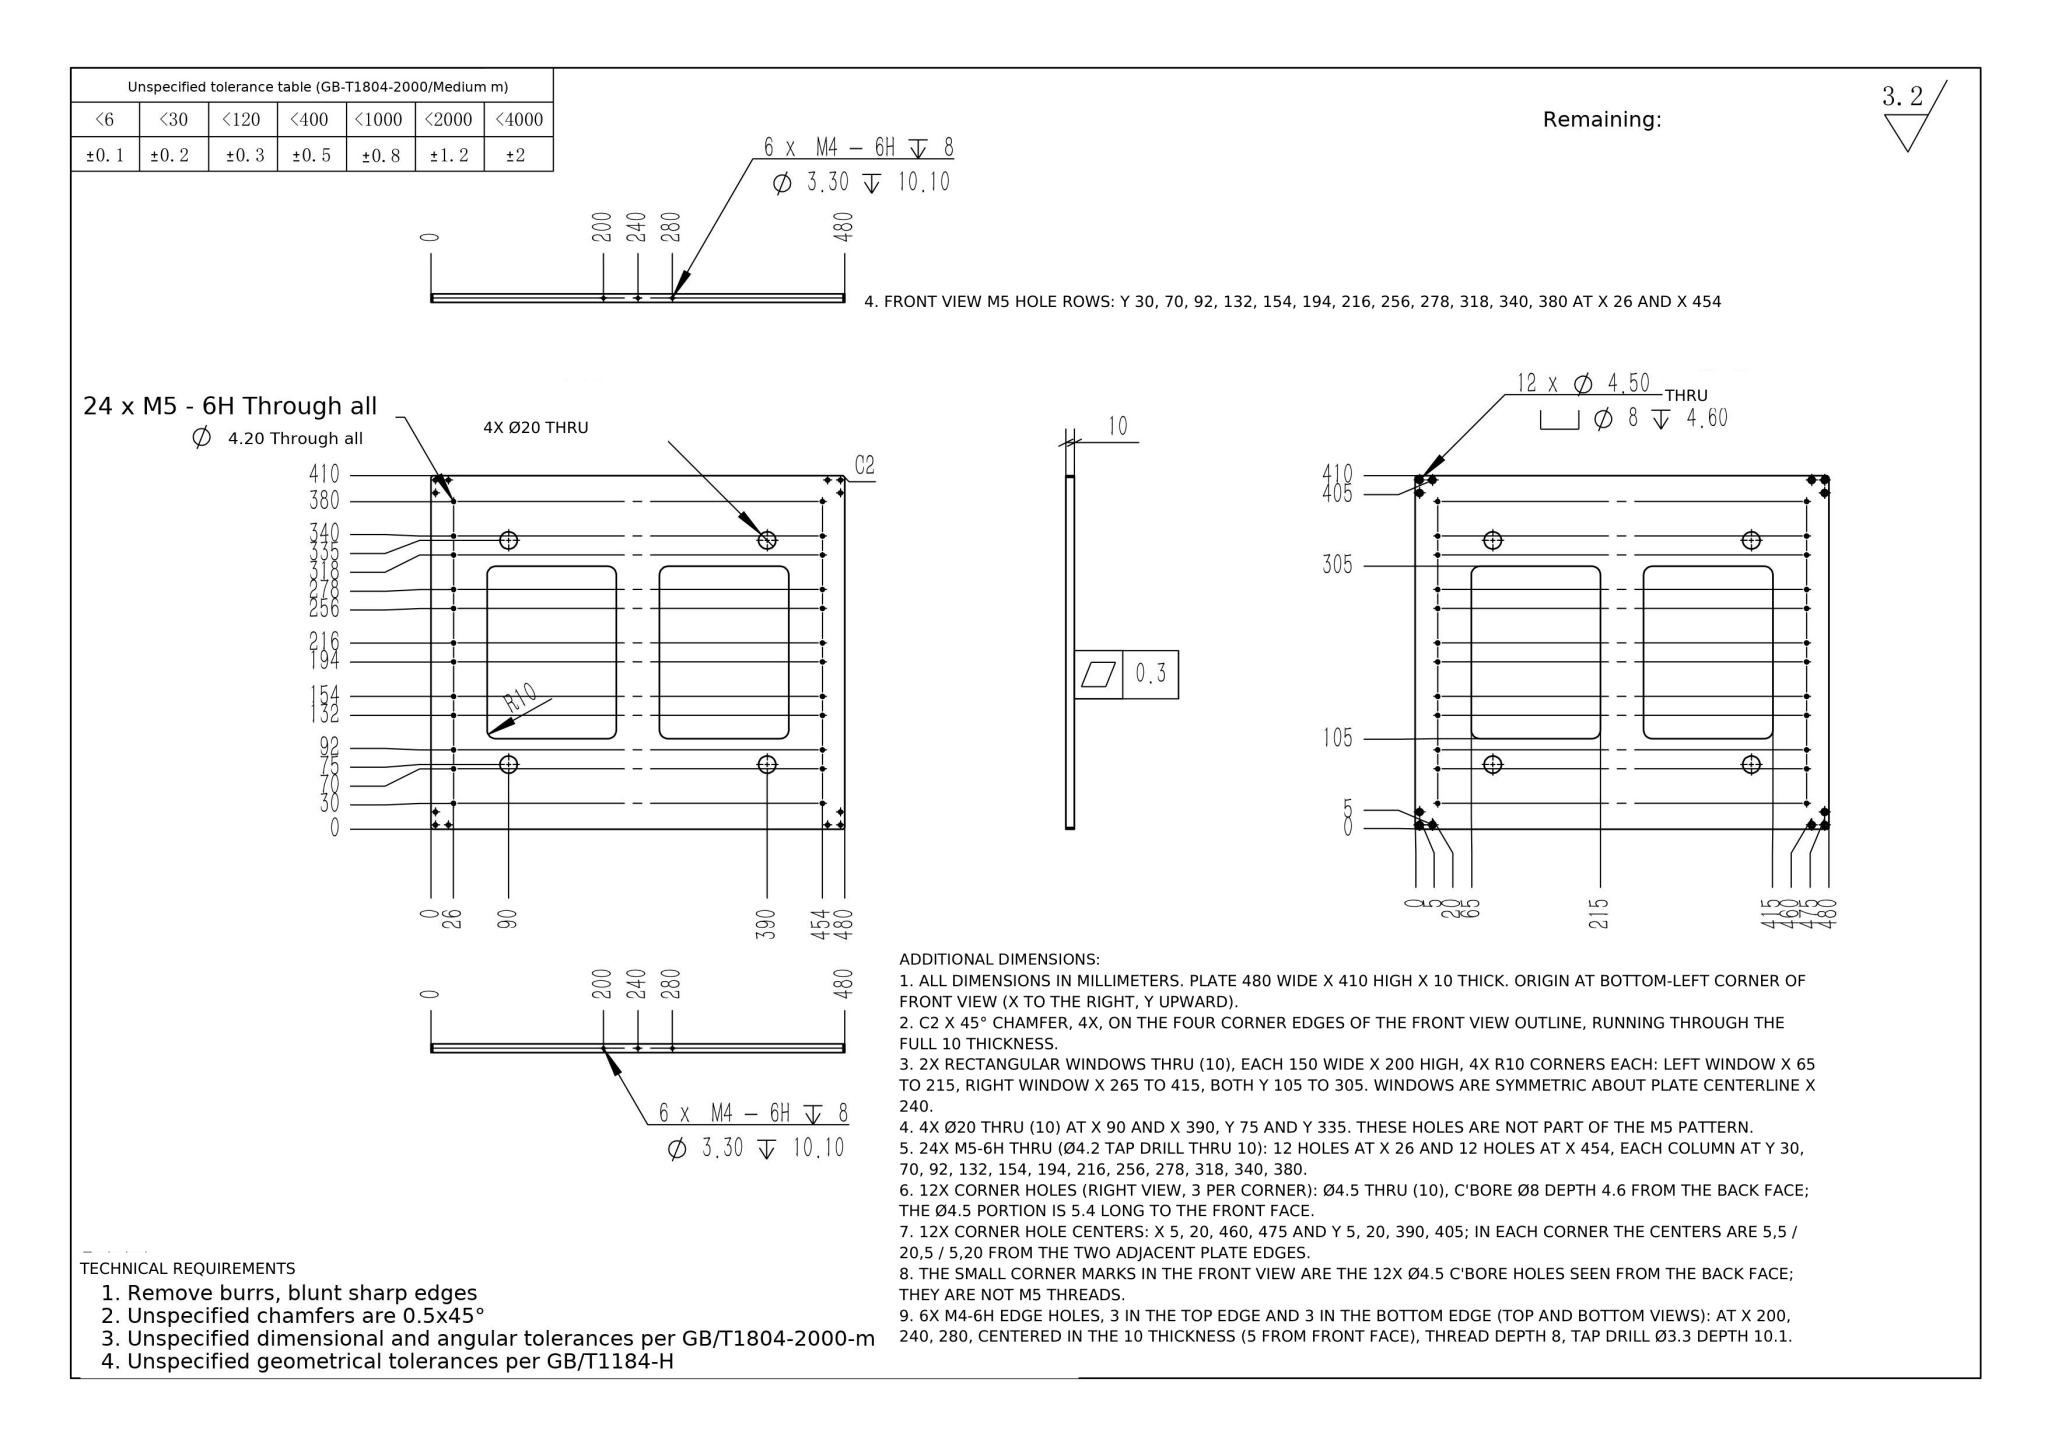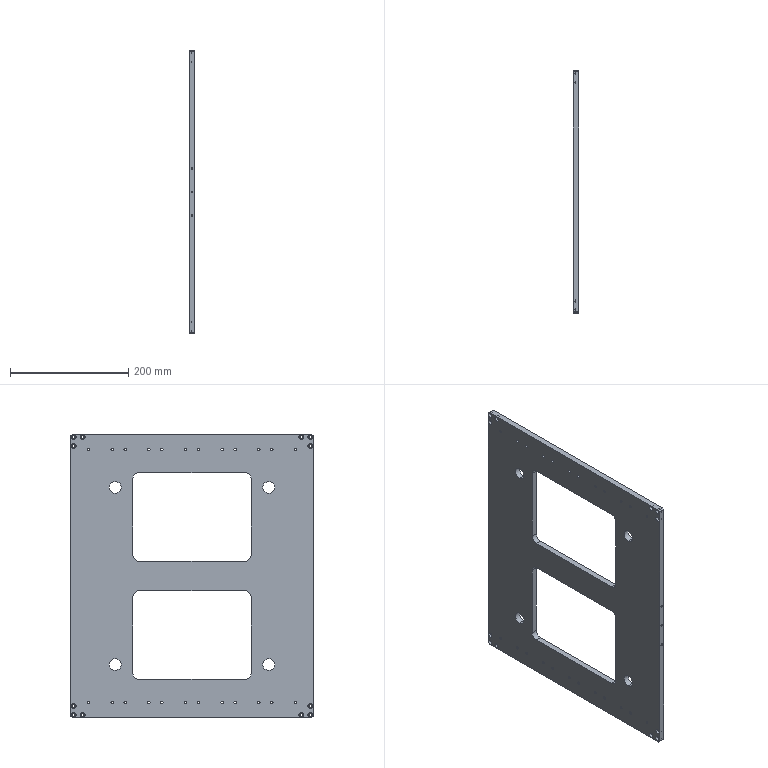Part | NX | mm | 1 solid | 166 faces | box 10 x 410 x 480 mm | volume 1349405 mm3 | cylinder 124 | plane 30 | cone 12 | commonest cylinder face diameters 4.2 x48 8 x24 4.5 x24 20 x16 3.3 x12